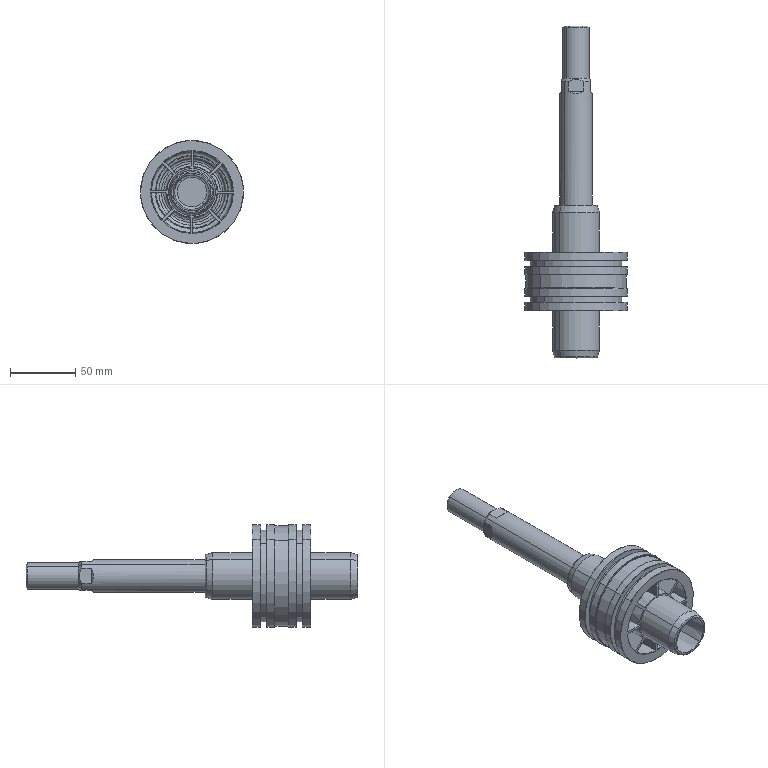Component | SolidWorks | AirTACCylinderFSC_80x75_S_FBAxis-1_FSC_80x75_S_FB_0_r-1 | 1 solid | 254 faces | volume 240889 mm3 | plane 84 | cone 74 | torus 74 | cylinder 22 | commonest cylinder face diameters 79 x8 36 x4 70 x4 76.9 x2 25 x2 20 x2